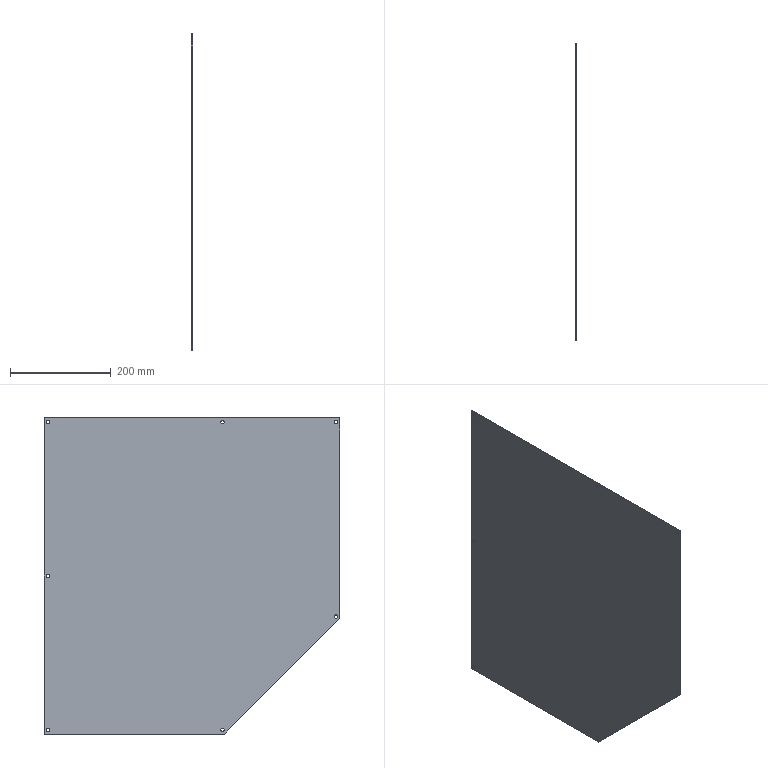Component | SolidWorks | RightSideWindow-1 | 1 solid | 21 faces | box 2 x 588 x 628 mm | volume 685089 mm3 | cylinder 14 | plane 7 | commonest cylinder face diameters 7 x14
build123d program:
from build123d import *

# Parameters (mm, degrees)
BOSS_EXTRUDE1_DEPTH = 2
SKETCH2_R           = 3.5
CUT_EXTRUDE1_DEPTH  = 2


with BuildPart() as part:
    # Sketch1 → Boss-Extrude1 (new body)
    with BuildSketch(Plane.XY):
        Polygon((-102.602, -465.965), (-102.602, 12.035), (-102.602, 122.035), (-48.577, 122.035), (525.398, 122.035), (525.398, -235.965), (295.398, -465.965), align=None)
    extrude(amount=BOSS_EXTRUDE1_DEPTH)

    # Sketch2 → Cut-Extrude1 (cut)
    with BuildSketch(Plane.XY.offset(2)):
        with Locations((517.398, 114.035)):
            Circle(SKETCH2_R)
        with Locations((517.398, -232.651)):
            Circle(SKETCH2_R)
        with Locations((292.085, -457.965)):
            Circle(SKETCH2_R)
        with Locations((-94.602, -457.965)):
            Circle(SKETCH2_R)
        with Locations((-94.602, -232.651)):
            Circle(SKETCH2_R)
        with Locations((-94.602, 114.035)):
            Circle(SKETCH2_R)
        with Locations((211.398, 114.035)):
            Circle(SKETCH2_R)
    extrude(amount=-CUT_EXTRUDE1_DEPTH, mode=Mode.SUBTRACT)


solid = part.part

# Placed as in the assembly
solid = solid.moved(Location((783.45, 328.531, 142.879), (0, 90, 0)))
STEP:
#1=COLOUR_RGB('',0.7922,0.8196,0.9333);
#2=FILL_AREA_STYLE_COLOUR('',#1);
#3=FILL_AREA_STYLE('',(#2));
#4=SURFACE_STYLE_FILL_AREA(#3);
#5=SURFACE_SIDE_STYLE('',(#4));
#6=SURFACE_STYLE_USAGE(.BOTH.,#5);
#7=PRESENTATION_STYLE_ASSIGNMENT((#6));
#8=CARTESIAN_POINT('',(30.845,17.424,-2.56));
#9=VERTEX_POINT('',#8);
#10=CARTESIAN_POINT('',(30.845,17.424,-2.835));
#11=VERTEX_POINT('',#10);
#12=CARTESIAN_POINT('',(30.845,17.424,-2.698));
#13=DIRECTION('',(1.,0.,0.));
#14=DIRECTION('',(0.,0.,-1.));
#15=AXIS2_PLACEMENT_3D('',#12,#13,#14);
#16=CIRCLE('',#15,0.1378);
#17=EDGE_CURVE('',#9,#11,#16,.T.);
#18=ORIENTED_EDGE('',*,*,#17,.F.);
#19=CARTESIAN_POINT('',(30.923,17.424,-2.56));
#20=VERTEX_POINT('',#19);
#21=CARTESIAN_POINT('',(30.845,17.424,-2.56));
#22=DIRECTION('',(1.,0.,0.));
#23=VECTOR('',#22,39.37);
#24=LINE('',#21,#23);
#25=EDGE_CURVE('',#9,#20,#24,.T.);
#26=ORIENTED_EDGE('',*,*,#25,.T.);
#27=CARTESIAN_POINT('',(30.923,17.424,-2.835));
#28=VERTEX_POINT('',#27);
#29=CARTESIAN_POINT('',(30.923,17.424,-2.698));
#30=DIRECTION('',(1.,0.,0.));
#31=DIRECTION('',(0.,0.,-1.));
#32=AXIS2_PLACEMENT_3D('',#29,#30,#31);
#33=CIRCLE('',#32,0.1378);
#34=EDGE_CURVE('',#20,#28,#33,.T.);
#35=ORIENTED_EDGE('',*,*,#34,.T.);
#36=CARTESIAN_POINT('',(30.845,17.424,-2.835));
#37=DIRECTION('',(1.,0.,0.));
#38=VECTOR('',#37,39.37);
#39=LINE('',#36,#38);
#40=EDGE_CURVE('',#11,#28,#39,.T.);
#41=ORIENTED_EDGE('',*,*,#40,.F.);
#42=EDGE_LOOP('',(#18,#26,#35,#41));
#43=FACE_OUTER_BOUND('',#42,.T.);
#44=CARTESIAN_POINT('',(30.845,17.424,-2.698));
#45=DIRECTION('',(1.,0.,0.));
#46=DIRECTION('',(0.,0.,-1.));
#47=AXIS2_PLACEMENT_3D('',#44,#45,#46);
#48=CYLINDRICAL_SURFACE('',#47,0.1378);
#49=ADVANCED_FACE('',(#43),#48,.F.);
#50=CARTESIAN_POINT('',(30.845,17.424,9.487));
#51=VERTEX_POINT('',#50);
#52=CARTESIAN_POINT('',(30.845,17.424,9.212));
#53=VERTEX_POINT('',#52);
#54=CARTESIAN_POINT('',(30.845,17.424,9.35));
#55=DIRECTION('',(1.,0.,0.));
#56=DIRECTION('',(0.,0.,-1.));
#57=AXIS2_PLACEMENT_3D('',#54,#55,#56);
#58=CIRCLE('',#57,0.1378);
#59=EDGE_CURVE('',#51,#53,#58,.T.);
#60=ORIENTED_EDGE('',*,*,#59,.F.);
#61=CARTESIAN_POINT('',(30.923,17.424,9.487));
#62=VERTEX_POINT('',#61);
#63=CARTESIAN_POINT('',(30.845,17.424,9.487));
#64=DIRECTION('',(1.,0.,0.));
#65=VECTOR('',#64,39.37);
#66=LINE('',#63,#65);
#67=EDGE_CURVE('',#51,#62,#66,.T.);
#68=ORIENTED_EDGE('',*,*,#67,.T.);
#69=CARTESIAN_POINT('',(30.923,17.424,9.212));
#70=VERTEX_POINT('',#69);
#71=CARTESIAN_POINT('',(30.923,17.424,9.35));
#72=DIRECTION('',(1.,0.,0.));
#73=DIRECTION('',(0.,0.,-1.));
#74=AXIS2_PLACEMENT_3D('',#71,#72,#73);
#75=CIRCLE('',#74,0.1378);
#76=EDGE_CURVE('',#62,#70,#75,.T.);
#77=ORIENTED_EDGE('',*,*,#76,.T.);
#78=CARTESIAN_POINT('',(30.845,17.424,9.212));
#79=DIRECTION('',(1.,0.,0.));
#80=VECTOR('',#79,39.37);
#81=LINE('',#78,#80);
#82=EDGE_CURVE('',#53,#70,#81,.T.);
#83=ORIENTED_EDGE('',*,*,#82,.F.);
#84=EDGE_LOOP('',(#60,#68,#77,#83));
#85=FACE_OUTER_BOUND('',#84,.T.);
#86=CARTESIAN_POINT('',(30.845,17.424,9.35));
#87=DIRECTION('',(1.,0.,0.));
#88=DIRECTION('',(0.,0.,-1.));
#89=AXIS2_PLACEMENT_3D('',#86,#87,#88);
#90=CYLINDRICAL_SURFACE('',#89,0.1378);
#91=ADVANCED_FACE('',(#85),#90,.F.);
#92=CARTESIAN_POINT('',(30.845,3.775,9.487));
#93=VERTEX_POINT('',#92);
#94=CARTESIAN_POINT('',(30.845,3.775,9.212));
#95=VERTEX_POINT('',#94);
#96=CARTESIAN_POINT('',(30.845,3.775,9.35));
#97=DIRECTION('',(1.,0.,0.));
#98=DIRECTION('',(0.,0.,-1.));
#99=AXIS2_PLACEMENT_3D('',#96,#97,#98);
#100=CIRCLE('',#99,0.1378);
#101=EDGE_CURVE('',#93,#95,#100,.T.);
#102=ORIENTED_EDGE('',*,*,#101,.F.);
#103=CARTESIAN_POINT('',(30.923,3.775,9.487));
#104=VERTEX_POINT('',#103);
#105=CARTESIAN_POINT('',(30.845,3.775,9.487));
#106=DIRECTION('',(1.,0.,0.));
#107=VECTOR('',#106,39.37);
#108=LINE('',#105,#107);
#109=EDGE_CURVE('',#93,#104,#108,.T.);
#110=ORIENTED_EDGE('',*,*,#109,.T.);
#111=CARTESIAN_POINT('',(30.923,3.775,9.212));
#112=VERTEX_POINT('',#111);
#113=CARTESIAN_POINT('',(30.923,3.775,9.35));
#114=DIRECTION('',(1.,0.,0.));
#115=DIRECTION('',(0.,0.,-1.));
#116=AXIS2_PLACEMENT_3D('',#113,#114,#115);
#117=CIRCLE('',#116,0.1378);
#118=EDGE_CURVE('',#104,#112,#117,.T.);
#119=ORIENTED_EDGE('',*,*,#118,.T.);
#120=CARTESIAN_POINT('',(30.845,3.775,9.212));
#121=DIRECTION('',(1.,0.,0.));
#122=VECTOR('',#121,39.37);
#123=LINE('',#120,#122);
#124=EDGE_CURVE('',#95,#112,#123,.T.);
#125=ORIENTED_EDGE('',*,*,#124,.F.);
#126=EDGE_LOOP('',(#102,#110,#119,#125));
#127=FACE_OUTER_BOUND('',#126,.T.);
#128=CARTESIAN_POINT('',(30.845,3.775,9.35));
#129=DIRECTION('',(1.,0.,0.));
#130=DIRECTION('',(0.,0.,-1.));
#131=AXIS2_PLACEMENT_3D('',#128,#129,#130);
#132=CYLINDRICAL_SURFACE('',#131,0.1378);
#133=ADVANCED_FACE('',(#127),#132,.F.);
#134=CARTESIAN_POINT('',(30.845,-5.096,9.487));
#135=VERTEX_POINT('',#134);
#136=CARTESIAN_POINT('',(30.845,-5.096,9.212));
#137=VERTEX_POINT('',#136);
#138=CARTESIAN_POINT('',(30.845,-5.096,9.35));
#139=DIRECTION('',(1.,0.,0.));
#140=DIRECTION('',(0.,0.,-1.));
#141=AXIS2_PLACEMENT_3D('',#138,#139,#140);
#142=CIRCLE('',#141,0.1378);
#143=EDGE_CURVE('',#135,#137,#142,.T.);
#144=ORIENTED_EDGE('',*,*,#143,.F.);
#145=CARTESIAN_POINT('',(30.923,-5.096,9.487));
#146=VERTEX_POINT('',#145);
#147=CARTESIAN_POINT('',(30.845,-5.096,9.487));
#148=DIRECTION('',(1.,0.,0.));
#149=VECTOR('',#148,39.37);
#150=LINE('',#147,#149);
#151=EDGE_CURVE('',#135,#146,#150,.T.);
#152=ORIENTED_EDGE('',*,*,#151,.T.);
#153=CARTESIAN_POINT('',(30.923,-5.096,9.212));
#154=VERTEX_POINT('',#153);
#155=CARTESIAN_POINT('',(30.923,-5.096,9.35));
#156=DIRECTION('',(1.,0.,0.));
#157=DIRECTION('',(0.,0.,-1.));
#158=AXIS2_PLACEMENT_3D('',#155,#156,#157);
#159=CIRCLE('',#158,0.1378);
#160=EDGE_CURVE('',#146,#154,#159,.T.);
#161=ORIENTED_EDGE('',*,*,#160,.T.);
#162=CARTESIAN_POINT('',(30.845,-5.096,9.212));
#163=DIRECTION('',(1.,0.,0.));
#164=VECTOR('',#163,39.37);
#165=LINE('',#162,#164);
#166=EDGE_CURVE('',#137,#154,#165,.T.);
#167=ORIENTED_EDGE('',*,*,#166,.F.);
#168=EDGE_LOOP('',(#144,#152,#161,#167));
#169=FACE_OUTER_BOUND('',#168,.T.);
#170=CARTESIAN_POINT('',(30.845,-5.096,9.35));
#171=DIRECTION('',(1.,0.,0.));
#172=DIRECTION('',(0.,0.,-1.));
#173=AXIS2_PLACEMENT_3D('',#170,#171,#172);
#174=CYLINDRICAL_SURFACE('',#173,0.1378);
#175=ADVANCED_FACE('',(#169),#174,.F.);
#176=CARTESIAN_POINT('',(30.845,-5.096,-5.736));
#177=VERTEX_POINT('',#176);
#178=CARTESIAN_POINT('',(30.845,-5.096,-6.012));
#179=VERTEX_POINT('',#178);
#180=CARTESIAN_POINT('',(30.845,-5.096,-5.874));
#181=DIRECTION('',(1.,0.,0.));
#182=DIRECTION('',(0.,0.,-1.));
#183=AXIS2_PLACEMENT_3D('',#180,#181,#182);
#184=CIRCLE('',#183,0.1378);
#185=EDGE_CURVE('',#177,#179,#184,.T.);
#186=ORIENTED_EDGE('',*,*,#185,.F.);
#187=CARTESIAN_POINT('',(30.923,-5.096,-5.736));
#188=VERTEX_POINT('',#187);
#189=CARTESIAN_POINT('',(30.845,-5.096,-5.736));
#190=DIRECTION('',(1.,0.,0.));
#191=VECTOR('',#190,39.37);
#192=LINE('',#189,#191);
#193=EDGE_CURVE('',#177,#188,#192,.T.);
#194=ORIENTED_EDGE('',*,*,#193,.T.);
#195=CARTESIAN_POINT('',(30.923,-5.096,-6.012));
#196=VERTEX_POINT('',#195);
#197=CARTESIAN_POINT('',(30.923,-5.096,-5.874));
#198=DIRECTION('',(1.,0.,0.));
#199=DIRECTION('',(0.,0.,-1.));
#200=AXIS2_PLACEMENT_3D('',#197,#198,#199);
#201=CIRCLE('',#200,0.1378);
#202=EDGE_CURVE('',#188,#196,#201,.T.);
#203=ORIENTED_EDGE('',*,*,#202,.T.);
#204=CARTESIAN_POINT('',(30.845,-5.096,-6.012));
#205=DIRECTION('',(1.,0.,0.));
#206=VECTOR('',#205,39.37);
#207=LINE('',#204,#206);
#208=EDGE_CURVE('',#179,#196,#207,.T.);
#209=ORIENTED_EDGE('',*,*,#208,.F.);
#210=EDGE_LOOP('',(#186,#194,#203,#209));
#211=FACE_OUTER_BOUND('',#210,.T.);
#212=CARTESIAN_POINT('',(30.845,-5.096,-5.874));
#213=DIRECTION('',(1.,0.,0.));
#214=DIRECTION('',(0.,0.,-1.));
#215=AXIS2_PLACEMENT_3D('',#212,#213,#214);
#216=CYLINDRICAL_SURFACE('',#215,0.1378);
#217=ADVANCED_FACE('',(#211),#216,.F.);
#218=CARTESIAN_POINT('',(30.845,3.775,-14.607));
#219=VERTEX_POINT('',#218);
#220=CARTESIAN_POINT('',(30.845,3.775,-14.883));
#221=VERTEX_POINT('',#220);
#222=CARTESIAN_POINT('',(30.845,3.775,-14.745));
#223=DIRECTION('',(1.,0.,0.));
#224=DIRECTION('',(0.,0.,-1.));
#225=AXIS2_PLACEMENT_3D('',#222,#223,#224);
#226=CIRCLE('',#225,0.1378);
#227=EDGE_CURVE('',#219,#221,#226,.T.);
#228=ORIENTED_EDGE('',*,*,#227,.F.);
#229=CARTESIAN_POINT('',(30.923,3.775,-14.607));
#230=VERTEX_POINT('',#229);
#231=CARTESIAN_POINT('',(30.845,3.775,-14.607));
#232=DIRECTION('',(1.,0.,0.));
#233=VECTOR('',#232,39.37);
#234=LINE('',#231,#233);
#235=EDGE_CURVE('',#219,#230,#234,.T.);
#236=ORIENTED_EDGE('',*,*,#235,.T.);
#237=CARTESIAN_POINT('',(30.923,3.775,-14.883));
#238=VERTEX_POINT('',#237);
#239=CARTESIAN_POINT('',(30.923,3.775,-14.745));
#240=DIRECTION('',(1.,0.,0.));
#241=DIRECTION('',(0.,0.,-1.));
#242=AXIS2_PLACEMENT_3D('',#239,#240,#241);
#243=CIRCLE('',#242,0.1378);
#244=EDGE_CURVE('',#230,#238,#243,.T.);
#245=ORIENTED_EDGE('',*,*,#244,.T.);
#246=CARTESIAN_POINT('',(30.845,3.775,-14.883));
#247=DIRECTION('',(1.,0.,0.));
#248=VECTOR('',#247,39.37);
#249=LINE('',#246,#248);
#250=EDGE_CURVE('',#221,#238,#249,.T.);
#251=ORIENTED_EDGE('',*,*,#250,.F.);
#252=EDGE_LOOP('',(#228,#236,#245,#251));
#253=FACE_OUTER_BOUND('',#252,.T.);
#254=CARTESIAN_POINT('',(30.845,3.775,-14.745));
#255=DIRECTION('',(1.,0.,0.));
#256=DIRECTION('',(0.,0.,-1.));
#257=AXIS2_PLACEMENT_3D('',#254,#255,#256);
#258=CYLINDRICAL_SURFACE('',#257,0.1378);
#259=ADVANCED_FACE('',(#253),#258,.F.);
#260=CARTESIAN_POINT('',(30.845,17.424,-14.607));
#261=VERTEX_POINT('',#260);
#262=CARTESIAN_POINT('',(30.845,17.424,-14.883));
#263=VERTEX_POINT('',#262);
#264=CARTESIAN_POINT('',(30.845,17.424,-14.745));
#265=DIRECTION('',(1.,0.,0.));
#266=DIRECTION('',(0.,0.,-1.));
#267=AXIS2_PLACEMENT_3D('',#264,#265,#266);
#268=CIRCLE('',#267,0.1378);
#269=EDGE_CURVE('',#261,#263,#268,.T.);
#270=ORIENTED_EDGE('',*,*,#269,.F.);
#271=CARTESIAN_POINT('',(30.923,17.424,-14.607));
#272=VERTEX_POINT('',#271);
#273=CARTESIAN_POINT('',(30.845,17.424,-14.607));
#274=DIRECTION('',(1.,0.,0.));
#275=VECTOR('',#274,39.37);
#276=LINE('',#273,#275);
#277=EDGE_CURVE('',#261,#272,#276,.T.);
#278=ORIENTED_EDGE('',*,*,#277,.T.);
#279=CARTESIAN_POINT('',(30.923,17.424,-14.883));
#280=VERTEX_POINT('',#279);
#281=CARTESIAN_POINT('',(30.923,17.424,-14.745));
#282=DIRECTION('',(1.,0.,0.));
#283=DIRECTION('',(0.,0.,-1.));
#284=AXIS2_PLACEMENT_3D('',#281,#282,#283);
#285=CIRCLE('',#284,0.1378);
#286=EDGE_CURVE('',#272,#280,#285,.T.);
#287=ORIENTED_EDGE('',*,*,#286,.T.);
#288=CARTESIAN_POINT('',(30.845,17.424,-14.883));
#289=DIRECTION('',(1.,0.,0.));
#290=VECTOR('',#289,39.37);
#291=LINE('',#288,#290);
#292=EDGE_CURVE('',#263,#280,#291,.T.);
#293=ORIENTED_EDGE('',*,*,#292,.F.);
#294=EDGE_LOOP('',(#270,#278,#287,#293));
#295=FACE_OUTER_BOUND('',#294,.T.);
#296=CARTESIAN_POINT('',(30.845,17.424,-14.745));
#297=DIRECTION('',(1.,0.,0.));
#298=DIRECTION('',(0.,0.,-1.));
#299=AXIS2_PLACEMENT_3D('',#296,#297,#298);
#300=CYLINDRICAL_SURFACE('',#299,0.1378);
#301=ADVANCED_FACE('',(#295),#300,.F.);
#302=CARTESIAN_POINT('',(30.845,-5.411,9.665));
#303=VERTEX_POINT('',#302);
#304=CARTESIAN_POINT('',(30.845,-5.411,-6.005));
#305=VERTEX_POINT('',#304);
#306=CARTESIAN_POINT('',(30.845,-5.411,-6.005));
#307=DIRECTION('',(0.,0.,-1.));
#308=VECTOR('',#307,39.37);
#309=LINE('',#306,#308);
#310=EDGE_CURVE('',#303,#305,#309,.T.);
#311=ORIENTED_EDGE('',*,*,#310,.T.);
#312=CARTESIAN_POINT('',(30.923,-5.411,-6.005));
#313=VERTEX_POINT('',#312);
#314=CARTESIAN_POINT('',(30.923,-5.411,-6.005));
#315=DIRECTION('',(-1.,-0.,-0.));
#316=VECTOR('',#315,39.37);
#317=LINE('',#314,#316);
#318=EDGE_CURVE('',#313,#305,#317,.T.);
#319=ORIENTED_EDGE('',*,*,#318,.F.);
#320=CARTESIAN_POINT('',(30.923,-5.411,9.665));
#321=VERTEX_POINT('',#320);
#322=CARTESIAN_POINT('',(30.923,-5.411,-6.005));
#323=DIRECTION('',(0.,0.,-1.));
#324=VECTOR('',#323,39.37);
#325=LINE('',#322,#324);
#326=EDGE_CURVE('',#321,#313,#325,.T.);
#327=ORIENTED_EDGE('',*,*,#326,.F.);
#328=CARTESIAN_POINT('',(30.923,-5.411,9.665));
#329=DIRECTION('',(-1.,-0.,-0.));
#330=VECTOR('',#329,39.37);
#331=LINE('',#328,#330);
#332=EDGE_CURVE('',#321,#303,#331,.T.);
#333=ORIENTED_EDGE('',*,*,#332,.T.);
#334=EDGE_LOOP('',(#311,#319,#327,#333));
#335=FACE_OUTER_BOUND('',#334,.T.);
#336=CARTESIAN_POINT('',(30.923,-5.411,-6.005));
#337=DIRECTION('',(-0.,1.,0.));
#338=DIRECTION('',(-0.,-0.,1.));
#339=AXIS2_PLACEMENT_3D('',#336,#337,#338);
#340=PLANE('',#339);
#341=ADVANCED_FACE('',(#335),#340,.F.);
#342=CARTESIAN_POINT('',(30.845,3.644,-15.06));
#343=VERTEX_POINT('',#342);
#344=CARTESIAN_POINT('',(30.845,-5.411,-6.005));
#345=DIRECTION('',(-0.,0.7071,-0.7071));
#346=VECTOR('',#345,39.37);
#347=LINE('',#344,#346);
#348=EDGE_CURVE('',#305,#343,#347,.T.);
#349=ORIENTED_EDGE('',*,*,#348,.T.);
#350=CARTESIAN_POINT('',(30.923,3.644,-15.06));
#351=VERTEX_POINT('',#350);
#352=CARTESIAN_POINT('',(30.923,3.644,-15.06));
#353=DIRECTION('',(-1.,-0.,-0.));
#354=VECTOR('',#353,39.37);
#355=LINE('',#352,#354);
#356=EDGE_CURVE('',#351,#343,#355,.T.);
#357=ORIENTED_EDGE('',*,*,#356,.F.);
#358=CARTESIAN_POINT('',(30.923,-5.411,-6.005));
#359=DIRECTION('',(-0.,0.7071,-0.7071));
#360=VECTOR('',#359,39.37);
#361=LINE('',#358,#360);
#362=EDGE_CURVE('',#313,#351,#361,.T.);
#363=ORIENTED_EDGE('',*,*,#362,.F.);
#364=ORIENTED_EDGE('',*,*,#318,.T.);
#365=EDGE_LOOP('',(#349,#357,#363,#364));
#366=FACE_OUTER_BOUND('',#365,.T.);
#367=CARTESIAN_POINT('',(30.923,-5.411,-6.005));
#368=DIRECTION('',(-0.,0.7071,0.7071));
#369=DIRECTION('',(0.,-0.7071,0.7071));
#370=AXIS2_PLACEMENT_3D('',#367,#368,#369);
#371=PLANE('',#370);
#372=ADVANCED_FACE('',(#366),#371,.F.);
#373=CARTESIAN_POINT('',(30.845,17.739,-15.06));
#374=VERTEX_POINT('',#373);
#375=CARTESIAN_POINT('',(30.845,17.739,-15.06));
#376=DIRECTION('',(-0.,1.,0.));
#377=VECTOR('',#376,39.37);
#378=LINE('',#375,#377);
#379=EDGE_CURVE('',#343,#374,#378,.T.);
#380=ORIENTED_EDGE('',*,*,#379,.T.);
#381=CARTESIAN_POINT('',(30.923,17.739,-15.06));
#382=VERTEX_POINT('',#381);
#383=CARTESIAN_POINT('',(30.923,17.739,-15.06));
#384=DIRECTION('',(-1.,-0.,-0.));
#385=VECTOR('',#384,39.37);
#386=LINE('',#383,#385);
#387=EDGE_CURVE('',#382,#374,#386,.T.);
#388=ORIENTED_EDGE('',*,*,#387,.F.);
#389=CARTESIAN_POINT('',(30.923,17.739,-15.06));
#390=DIRECTION('',(-0.,1.,0.));
#391=VECTOR('',#390,39.37);
#392=LINE('',#389,#391);
#393=EDGE_CURVE('',#351,#382,#392,.T.);
#394=ORIENTED_EDGE('',*,*,#393,.F.);
#395=ORIENTED_EDGE('',*,*,#356,.T.);
#396=EDGE_LOOP('',(#380,#388,#394,#395));
#397=FACE_OUTER_BOUND('',#396,.T.);
#398=CARTESIAN_POINT('',(30.923,17.739,-15.06));
#399=DIRECTION('',(-0.,0.,1.));
#400=DIRECTION('',(1.,0.,0.));
#401=AXIS2_PLACEMENT_3D('',#398,#399,#400);
#402=PLANE('',#401);
#403=ADVANCED_FACE('',(#397),#402,.F.);
#404=CARTESIAN_POINT('',(30.845,17.739,9.665));
#405=VERTEX_POINT('',#404);
#406=CARTESIAN_POINT('',(30.845,17.739,7.538));
#407=DIRECTION('',(-0.,-0.,1.));
#408=VECTOR('',#407,39.37);
#409=LINE('',#406,#408);
#410=EDGE_CURVE('',#374,#405,#409,.T.);
#411=ORIENTED_EDGE('',*,*,#410,.T.);
#412=CARTESIAN_POINT('',(30.923,17.739,9.665));
#413=VERTEX_POINT('',#412);
#414=CARTESIAN_POINT('',(30.923,17.739,9.665));
#415=DIRECTION('',(-1.,-0.,-0.));
#416=VECTOR('',#415,39.37);
#417=LINE('',#414,#416);
#418=EDGE_CURVE('',#413,#405,#417,.T.);
#419=ORIENTED_EDGE('',*,*,#418,.F.);
#420=CARTESIAN_POINT('',(30.923,17.739,7.538));
#421=DIRECTION('',(-0.,0.,1.));
#422=VECTOR('',#421,39.37);
#423=LINE('',#420,#422);
#424=EDGE_CURVE('',#382,#413,#423,.T.);
#425=ORIENTED_EDGE('',*,*,#424,.F.);
#426=ORIENTED_EDGE('',*,*,#387,.T.);
#427=EDGE_LOOP('',(#411,#419,#425,#426));
#428=FACE_OUTER_BOUND('',#427,.T.);
#429=CARTESIAN_POINT('',(30.923,17.739,7.538));
#430=DIRECTION('',(0.,-1.,-0.));
#431=DIRECTION('',(0.,0.,-1.));
#432=AXIS2_PLACEMENT_3D('',#429,#430,#431);
#433=PLANE('',#432);
#434=ADVANCED_FACE('',(#428),#433,.F.);
#435=CARTESIAN_POINT('',(30.845,-5.411,9.665));
#436=DIRECTION('',(0.,-1.,-0.));
#437=VECTOR('',#436,39.37);
#438=LINE('',#435,#437);
#439=EDGE_CURVE('',#405,#303,#438,.T.);
#440=ORIENTED_EDGE('',*,*,#439,.T.);
#441=ORIENTED_EDGE('',*,*,#332,.F.);
#442=CARTESIAN_POINT('',(30.923,17.739,9.665));
#443=DIRECTION('',(0.,-1.,-0.));
#444=VECTOR('',#443,39.37);
#445=LINE('',#442,#444);
#446=EDGE_CURVE('',#413,#321,#445,.T.);
#447=ORIENTED_EDGE('',*,*,#446,.F.);
#448=ORIENTED_EDGE('',*,*,#418,.T.);
#449=EDGE_LOOP('',(#440,#441,#447,#448));
#450=FACE_OUTER_BOUND('',#449,.T.);
#451=CARTESIAN_POINT('',(30.923,-5.411,9.665));
#452=DIRECTION('',(0.,0.,-1.));
#453=DIRECTION('',(-0.,1.,0.));
#454=AXIS2_PLACEMENT_3D('',#451,#452,#453);
#455=PLANE('',#454);
#456=ADVANCED_FACE('',(#450),#455,.F.);
#457=CARTESIAN_POINT('',(30.923,17.424,-2.698));
#458=DIRECTION('',(1.,0.,0.));
#459=DIRECTION('',(0.,0.,-1.));
#460=AXIS2_PLACEMENT_3D('',#457,#458,#459);
#461=CIRCLE('',#460,0.1378);
#462=EDGE_CURVE('',#28,#20,#461,.T.);
#463=ORIENTED_EDGE('',*,*,#462,.F.);
#464=ORIENTED_EDGE('',*,*,#34,.F.);
#465=EDGE_LOOP('',(#463,#464));
#466=FACE_BOUND('',#465,.T.);
#467=CARTESIAN_POINT('',(30.923,17.424,9.35));
#468=DIRECTION('',(1.,0.,0.));
#469=DIRECTION('',(0.,0.,-1.));
#470=AXIS2_PLACEMENT_3D('',#467,#468,#469);
#471=CIRCLE('',#470,0.1378);
#472=EDGE_CURVE('',#70,#62,#471,.T.);
#473=ORIENTED_EDGE('',*,*,#472,.F.);
#474=ORIENTED_EDGE('',*,*,#76,.F.);
#475=EDGE_LOOP('',(#473,#474));
#476=FACE_BOUND('',#475,.T.);
#477=CARTESIAN_POINT('',(30.923,3.775,9.35));
#478=DIRECTION('',(1.,0.,0.));
#479=DIRECTION('',(0.,0.,-1.));
#480=AXIS2_PLACEMENT_3D('',#477,#478,#479);
#481=CIRCLE('',#480,0.1378);
#482=EDGE_CURVE('',#112,#104,#481,.T.);
#483=ORIENTED_EDGE('',*,*,#482,.F.);
#484=ORIENTED_EDGE('',*,*,#118,.F.);
#485=EDGE_LOOP('',(#483,#484));
#486=FACE_BOUND('',#485,.T.);
#487=CARTESIAN_POINT('',(30.923,-5.096,9.35));
#488=DIRECTION('',(1.,0.,0.));
#489=DIRECTION('',(0.,0.,-1.));
#490=AXIS2_PLACEMENT_3D('',#487,#488,#489);
#491=CIRCLE('',#490,0.1378);
#492=EDGE_CURVE('',#154,#146,#491,.T.);
#493=ORIENTED_EDGE('',*,*,#492,.F.);
#494=ORIENTED_EDGE('',*,*,#160,.F.);
#495=EDGE_LOOP('',(#493,#494));
#496=FACE_BOUND('',#495,.T.);
#497=CARTESIAN_POINT('',(30.923,-5.096,-5.874));
#498=DIRECTION('',(1.,0.,0.));
#499=DIRECTION('',(0.,0.,-1.));
#500=AXIS2_PLACEMENT_3D('',#497,#498,#499);
#501=CIRCLE('',#500,0.1378);
#502=EDGE_CURVE('',#196,#188,#501,.T.);
#503=ORIENTED_EDGE('',*,*,#502,.F.);
#504=ORIENTED_EDGE('',*,*,#202,.F.);
#505=EDGE_LOOP('',(#503,#504));
#506=FACE_BOUND('',#505,.T.);
#507=CARTESIAN_POINT('',(30.923,3.775,-14.745));
#508=DIRECTION('',(1.,0.,0.));
#509=DIRECTION('',(0.,0.,-1.));
#510=AXIS2_PLACEMENT_3D('',#507,#508,#509);
#511=CIRCLE('',#510,0.1378);
#512=EDGE_CURVE('',#238,#230,#511,.T.);
#513=ORIENTED_EDGE('',*,*,#512,.F.);
#514=ORIENTED_EDGE('',*,*,#244,.F.);
#515=EDGE_LOOP('',(#513,#514));
#516=FACE_BOUND('',#515,.T.);
#517=CARTESIAN_POINT('',(30.923,17.424,-14.745));
#518=DIRECTION('',(1.,0.,0.));
#519=DIRECTION('',(0.,0.,-1.));
#520=AXIS2_PLACEMENT_3D('',#517,#518,#519);
#521=CIRCLE('',#520,0.1378);
#522=EDGE_CURVE('',#280,#272,#521,.T.);
#523=ORIENTED_EDGE('',*,*,#522,.F.);
#524=ORIENTED_EDGE('',*,*,#286,.F.);
#525=EDGE_LOOP('',(#523,#524));
#526=FACE_BOUND('',#525,.T.);
#527=ORIENTED_EDGE('',*,*,#326,.T.);
#528=ORIENTED_EDGE('',*,*,#362,.T.);
#529=ORIENTED_EDGE('',*,*,#393,.T.);
#530=ORIENTED_EDGE('',*,*,#424,.T.);
#531=ORIENTED_EDGE('',*,*,#446,.T.);
#532=EDGE_LOOP('',(#527,#528,#529,#530,#531));
#533=FACE_OUTER_BOUND('',#532,.T.);
#534=CARTESIAN_POINT('',(30.923,12.934,5.625));
#535=DIRECTION('',(-1.,-0.,-0.));
#536=DIRECTION('',(-0.,0.,1.));
#537=AXIS2_PLACEMENT_3D('',#534,#535,#536);
#538=PLANE('',#537);
#539=ADVANCED_FACE('',(#466,#476,#486,#496,#506,#516,#526,#533),#538,.F.);
#540=CARTESIAN_POINT('',(30.845,17.424,-2.698));
#541=DIRECTION('',(1.,0.,0.));
#542=DIRECTION('',(0.,0.,-1.));
#543=AXIS2_PLACEMENT_3D('',#540,#541,#542);
#544=CIRCLE('',#543,0.1378);
#545=EDGE_CURVE('',#11,#9,#544,.T.);
#546=ORIENTED_EDGE('',*,*,#545,.T.);
#547=ORIENTED_EDGE('',*,*,#17,.T.);
#548=EDGE_LOOP('',(#546,#547));
#549=FACE_BOUND('',#548,.T.);
#550=CARTESIAN_POINT('',(30.845,17.424,9.35));
#551=DIRECTION('',(1.,0.,0.));
#552=DIRECTION('',(0.,0.,-1.));
#553=AXIS2_PLACEMENT_3D('',#550,#551,#552);
#554=CIRCLE('',#553,0.1378);
#555=EDGE_CURVE('',#53,#51,#554,.T.);
#556=ORIENTED_EDGE('',*,*,#555,.T.);
#557=ORIENTED_EDGE('',*,*,#59,.T.);
#558=EDGE_LOOP('',(#556,#557));
#559=FACE_BOUND('',#558,.T.);
#560=CARTESIAN_POINT('',(30.845,3.775,9.35));
#561=DIRECTION('',(1.,0.,0.));
#562=DIRECTION('',(0.,0.,-1.));
#563=AXIS2_PLACEMENT_3D('',#560,#561,#562);
#564=CIRCLE('',#563,0.1378);
#565=EDGE_CURVE('',#95,#93,#564,.T.);
#566=ORIENTED_EDGE('',*,*,#565,.T.);
#567=ORIENTED_EDGE('',*,*,#101,.T.);
#568=EDGE_LOOP('',(#566,#567));
#569=FACE_BOUND('',#568,.T.);
#570=CARTESIAN_POINT('',(30.845,-5.096,9.35));
#571=DIRECTION('',(1.,0.,0.));
#572=DIRECTION('',(0.,0.,-1.));
#573=AXIS2_PLACEMENT_3D('',#570,#571,#572);
#574=CIRCLE('',#573,0.1378);
#575=EDGE_CURVE('',#137,#135,#574,.T.);
#576=ORIENTED_EDGE('',*,*,#575,.T.);
#577=ORIENTED_EDGE('',*,*,#143,.T.);
#578=EDGE_LOOP('',(#576,#577));
#579=FACE_BOUND('',#578,.T.);
#580=CARTESIAN_POINT('',(30.845,-5.096,-5.874));
#581=DIRECTION('',(1.,0.,0.));
#582=DIRECTION('',(0.,0.,-1.));
#583=AXIS2_PLACEMENT_3D('',#580,#581,#582);
#584=CIRCLE('',#583,0.1378);
#585=EDGE_CURVE('',#179,#177,#584,.T.);
#586=ORIENTED_EDGE('',*,*,#585,.T.);
#587=ORIENTED_EDGE('',*,*,#185,.T.);
#588=EDGE_LOOP('',(#586,#587));
#589=FACE_BOUND('',#588,.T.);
#590=CARTESIAN_POINT('',(30.845,3.775,-14.745));
#591=DIRECTION('',(1.,0.,0.));
#592=DIRECTION('',(0.,0.,-1.));
#593=AXIS2_PLACEMENT_3D('',#590,#591,#592);
#594=CIRCLE('',#593,0.1378);
#595=EDGE_CURVE('',#221,#219,#594,.T.);
#596=ORIENTED_EDGE('',*,*,#595,.T.);
#597=ORIENTED_EDGE('',*,*,#227,.T.);
#598=EDGE_LOOP('',(#596,#597));
#599=FACE_BOUND('',#598,.T.);
#600=CARTESIAN_POINT('',(30.845,17.424,-14.745));
#601=DIRECTION('',(1.,0.,0.));
#602=DIRECTION('',(0.,0.,-1.));
#603=AXIS2_PLACEMENT_3D('',#600,#601,#602);
#604=CIRCLE('',#603,0.1378);
#605=EDGE_CURVE('',#263,#261,#604,.T.);
#606=ORIENTED_EDGE('',*,*,#605,.T.);
#607=ORIENTED_EDGE('',*,*,#269,.T.);
#608=EDGE_LOOP('',(#606,#607));
#609=FACE_BOUND('',#608,.T.);
#610=ORIENTED_EDGE('',*,*,#310,.F.);
#611=ORIENTED_EDGE('',*,*,#439,.F.);
#612=ORIENTED_EDGE('',*,*,#410,.F.);
#613=ORIENTED_EDGE('',*,*,#379,.F.);
#614=ORIENTED_EDGE('',*,*,#348,.F.);
#615=EDGE_LOOP('',(#610,#611,#612,#613,#614));
#616=FACE_OUTER_BOUND('',#615,.T.);
#617=CARTESIAN_POINT('',(30.845,12.934,5.625));
#618=DIRECTION('',(-1.,-0.,-0.));
#619=DIRECTION('',(-0.,0.,1.));
#620=AXIS2_PLACEMENT_3D('',#617,#618,#619);
#621=PLANE('',#620);
#622=ADVANCED_FACE('',(#549,#559,#569,#579,#589,#599,#609,#616),#621,.T.);
#623=ORIENTED_EDGE('',*,*,#277,.F.);
#624=ORIENTED_EDGE('',*,*,#605,.F.);
#625=ORIENTED_EDGE('',*,*,#292,.T.);
#626=ORIENTED_EDGE('',*,*,#522,.T.);
#627=EDGE_LOOP('',(#623,#624,#625,#626));
#628=FACE_OUTER_BOUND('',#627,.T.);
#629=CARTESIAN_POINT('',(30.845,17.424,-14.745));
#630=DIRECTION('',(1.,0.,0.));
#631=DIRECTION('',(0.,0.,-1.));
#632=AXIS2_PLACEMENT_3D('',#629,#630,#631);
#633=CYLINDRICAL_SURFACE('',#632,0.1378);
#634=ADVANCED_FACE('',(#628),#633,.F.);
#635=ORIENTED_EDGE('',*,*,#235,.F.);
#636=ORIENTED_EDGE('',*,*,#595,.F.);
#637=ORIENTED_EDGE('',*,*,#250,.T.);
#638=ORIENTED_EDGE('',*,*,#512,.T.);
#639=EDGE_LOOP('',(#635,#636,#637,#638));
#640=FACE_OUTER_BOUND('',#639,.T.);
#641=CARTESIAN_POINT('',(30.845,3.775,-14.745));
#642=DIRECTION('',(1.,0.,0.));
#643=DIRECTION('',(0.,0.,-1.));
#644=AXIS2_PLACEMENT_3D('',#641,#642,#643);
#645=CYLINDRICAL_SURFACE('',#644,0.1378);
#646=ADVANCED_FACE('',(#640),#645,.F.);
#647=ORIENTED_EDGE('',*,*,#193,.F.);
#648=ORIENTED_EDGE('',*,*,#585,.F.);
#649=ORIENTED_EDGE('',*,*,#208,.T.);
#650=ORIENTED_EDGE('',*,*,#502,.T.);
#651=EDGE_LOOP('',(#647,#648,#649,#650));
#652=FACE_OUTER_BOUND('',#651,.T.);
#653=CARTESIAN_POINT('',(30.845,-5.096,-5.874));
#654=DIRECTION('',(1.,0.,0.));
#655=DIRECTION('',(0.,0.,-1.));
#656=AXIS2_PLACEMENT_3D('',#653,#654,#655);
#657=CYLINDRICAL_SURFACE('',#656,0.1378);
#658=ADVANCED_FACE('',(#652),#657,.F.);
#659=ORIENTED_EDGE('',*,*,#151,.F.);
#660=ORIENTED_EDGE('',*,*,#575,.F.);
#661=ORIENTED_EDGE('',*,*,#166,.T.);
#662=ORIENTED_EDGE('',*,*,#492,.T.);
#663=EDGE_LOOP('',(#659,#660,#661,#662));
#664=FACE_OUTER_BOUND('',#663,.T.);
#665=CARTESIAN_POINT('',(30.845,-5.096,9.35));
#666=DIRECTION('',(1.,0.,0.));
#667=DIRECTION('',(0.,0.,-1.));
#668=AXIS2_PLACEMENT_3D('',#665,#666,#667);
#669=CYLINDRICAL_SURFACE('',#668,0.1378);
#670=ADVANCED_FACE('',(#664),#669,.F.);
#671=ORIENTED_EDGE('',*,*,#109,.F.);
#672=ORIENTED_EDGE('',*,*,#565,.F.);
#673=ORIENTED_EDGE('',*,*,#124,.T.);
#674=ORIENTED_EDGE('',*,*,#482,.T.);
#675=EDGE_LOOP('',(#671,#672,#673,#674));
#676=FACE_OUTER_BOUND('',#675,.T.);
#677=CARTESIAN_POINT('',(30.845,3.775,9.35));
#678=DIRECTION('',(1.,0.,0.));
#679=DIRECTION('',(0.,0.,-1.));
#680=AXIS2_PLACEMENT_3D('',#677,#678,#679);
#681=CYLINDRICAL_SURFACE('',#680,0.1378);
#682=ADVANCED_FACE('',(#676),#681,.F.);
#683=ORIENTED_EDGE('',*,*,#67,.F.);
#684=ORIENTED_EDGE('',*,*,#555,.F.);
#685=ORIENTED_EDGE('',*,*,#82,.T.);
#686=ORIENTED_EDGE('',*,*,#472,.T.);
#687=EDGE_LOOP('',(#683,#684,#685,#686));
#688=FACE_OUTER_BOUND('',#687,.T.);
#689=CARTESIAN_POINT('',(30.845,17.424,9.35));
#690=DIRECTION('',(1.,0.,0.));
#691=DIRECTION('',(0.,0.,-1.));
#692=AXIS2_PLACEMENT_3D('',#689,#690,#691);
#693=CYLINDRICAL_SURFACE('',#692,0.1378);
#694=ADVANCED_FACE('',(#688),#693,.F.);
#695=ORIENTED_EDGE('',*,*,#25,.F.);
#696=ORIENTED_EDGE('',*,*,#545,.F.);
#697=ORIENTED_EDGE('',*,*,#40,.T.);
#698=ORIENTED_EDGE('',*,*,#462,.T.);
#699=EDGE_LOOP('',(#695,#696,#697,#698));
#700=FACE_OUTER_BOUND('',#699,.T.);
#701=CARTESIAN_POINT('',(30.845,17.424,-2.698));
#702=DIRECTION('',(1.,0.,0.));
#703=DIRECTION('',(0.,0.,-1.));
#704=AXIS2_PLACEMENT_3D('',#701,#702,#703);
#705=CYLINDRICAL_SURFACE('',#704,0.1378);
#706=ADVANCED_FACE('',(#700),#705,.F.);
#707=CLOSED_SHELL('',(#49,#91,#133,#175,#217,#259,#301,#341,#372,#403,#434,#456,#539,#622,#634,#646,#658,#670,#682,#694,#706));
#708=MANIFOLD_SOLID_BREP('',#707);
#709=STYLED_ITEM('',(#7),#708);
#710=(LENGTH_UNIT()NAMED_UNIT(*)SI_UNIT($,.METRE.));
#711=LENGTH_MEASURE_WITH_UNIT(LENGTH_MEASURE(0.0254),#710);
#712=DIMENSIONAL_EXPONENTS(1.,0.,0.,0.,0.,0.,0.);
#713=(CONVERSION_BASED_UNIT('',#711)LENGTH_UNIT()NAMED_UNIT(#712));
#714=UNCERTAINTY_MEASURE_WITH_UNIT(LENGTH_MEASURE(0.00001),#713,'','');
#715=(NAMED_UNIT(*)PLANE_ANGLE_UNIT()SI_UNIT($,.RADIAN.));
#716=(NAMED_UNIT(*)SI_UNIT($,.STERADIAN.)SOLID_ANGLE_UNIT());
#717=(GEOMETRIC_REPRESENTATION_CONTEXT(3)GLOBAL_UNCERTAINTY_ASSIGNED_CONTEXT((#714))GLOBAL_UNIT_ASSIGNED_CONTEXT((#713,#715,#716))REPRESENTATION_CONTEXT('',''));
#718=MECHANICAL_DESIGN_GEOMETRIC_PRESENTATION_REPRESENTATION('',(#709),#717);
#719=CARTESIAN_POINT('',(0.,0.,0.));
#720=DIRECTION('',(0.,0.,1.));
#721=DIRECTION('',(1.,0.,0.));
#722=AXIS2_PLACEMENT_3D('',#719,#720,#721);
#723=(LENGTH_UNIT()NAMED_UNIT(*)SI_UNIT($,.METRE.));
#724=LENGTH_MEASURE_WITH_UNIT(LENGTH_MEASURE(0.0254),#723);
#725=DIMENSIONAL_EXPONENTS(1.,0.,0.,0.,0.,0.,0.);
#726=(CONVERSION_BASED_UNIT('',#724)LENGTH_UNIT()NAMED_UNIT(#725));
#727=UNCERTAINTY_MEASURE_WITH_UNIT(LENGTH_MEASURE(0.00001),#726,'','');
#728=(NAMED_UNIT(*)PLANE_ANGLE_UNIT()SI_UNIT($,.RADIAN.));
#729=(NAMED_UNIT(*)SI_UNIT($,.STERADIAN.)SOLID_ANGLE_UNIT());
#730=(GEOMETRIC_REPRESENTATION_CONTEXT(3)GLOBAL_UNCERTAINTY_ASSIGNED_CONTEXT((#727))GLOBAL_UNIT_ASSIGNED_CONTEXT((#726,#728,#729))REPRESENTATION_CONTEXT('',''));
#731=ADVANCED_BREP_SHAPE_REPRESENTATION('',(#708,#722),#730);
#732=PRESENTATION_LAYER_ASSIGNMENT('','',(#709));